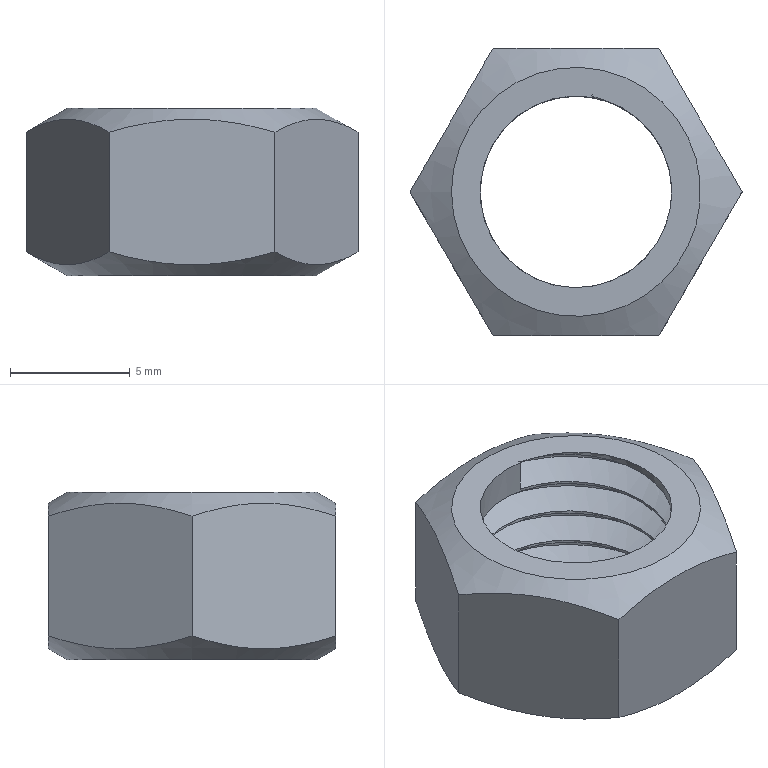Component | NX | NUT_M8 | 1 solid | 15 faces | volume 399 mm3 | plane 9 | cylinder 2 | cone 2 | spline 2 | commonest cylinder face diameters 8 x1 10 x1